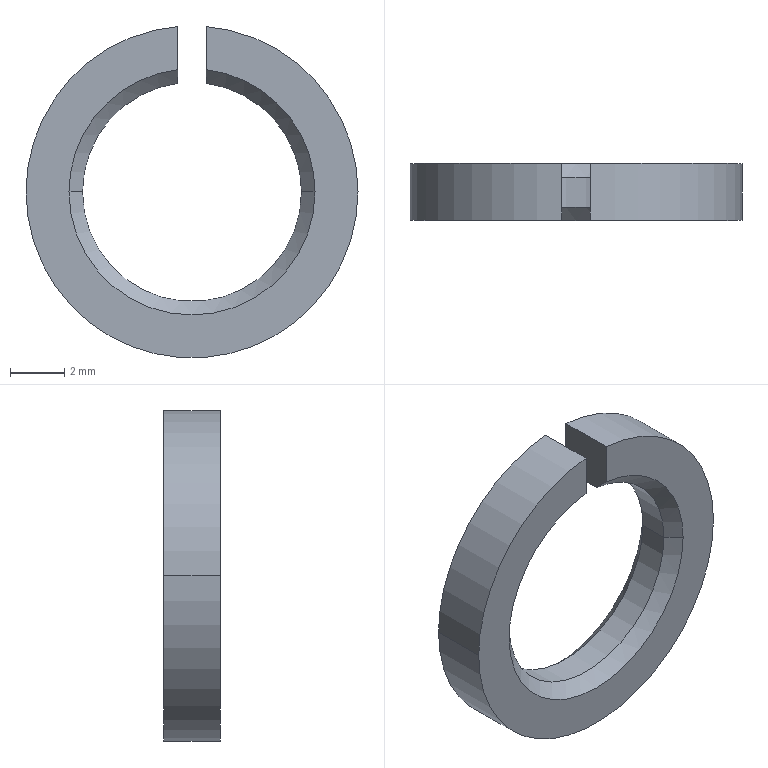Component | SolidWorks | StandardTypeSpringWasher(Assembly)8_2.1[GB_T93-1987]-1 | 1 solid | 16 faces | box 12.28 x 2.1 x 12.25 mm | volume 129 mm3 | cone 6 | cylinder 6 | plane 4 | commonest cylinder face diameters 8.1 x3 12.277 x3
build123d program:
from build123d import *

# Parameters (mm, degrees)
EXTRUDE1_DEPTH = 2.1
CHAMFER1_SIZE  = 0.5


with BuildPart() as part:
    # Sketch1 → Extrude1 (new body)
    with BuildSketch(Plane.XY):
        with BuildLine():
            Line((-0.525, 6.116), (-0.525, 4.016))
            ThreePointArc((-0.525, 4.016), (0, -4.05), (0.525, 4.016))
            Line((0.525, 4.016), (0.525, 6.116))
            ThreePointArc((0.525, 6.116), (0, -6.138), (-0.525, 6.116))
        make_face()
    extrude(amount=EXTRUDE1_DEPTH)

    # Chamfer1
    chamfer1_edges = [part.edges().sort_by_distance(p)[0] for p in [
        (0, -4.05, 2.1),
        (0, -4.05, 0),
    ]]
    chamfer(chamfer1_edges, length=CHAMFER1_SIZE)


solid = part.part

# Placed as in the assembly
solid = solid.moved(Location((-40.006, 37.7, 26), (90, 0, 0)))